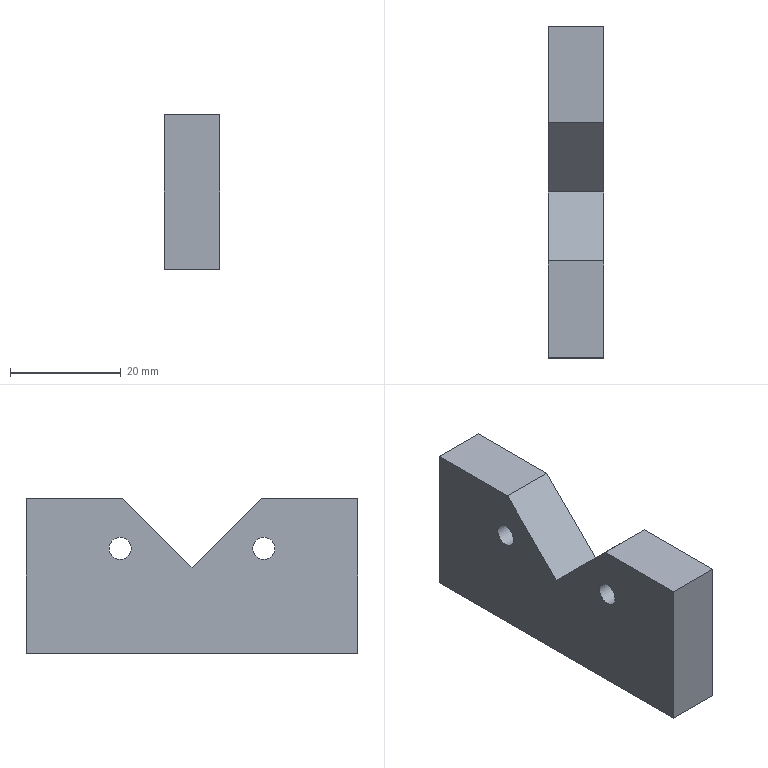Component | NX | FRONT_BRACKET | 1 solid | 19 faces | volume 13769 mm3 | plane 13 | cylinder 6 | commonest cylinder face diameters 5 x4 4 x2